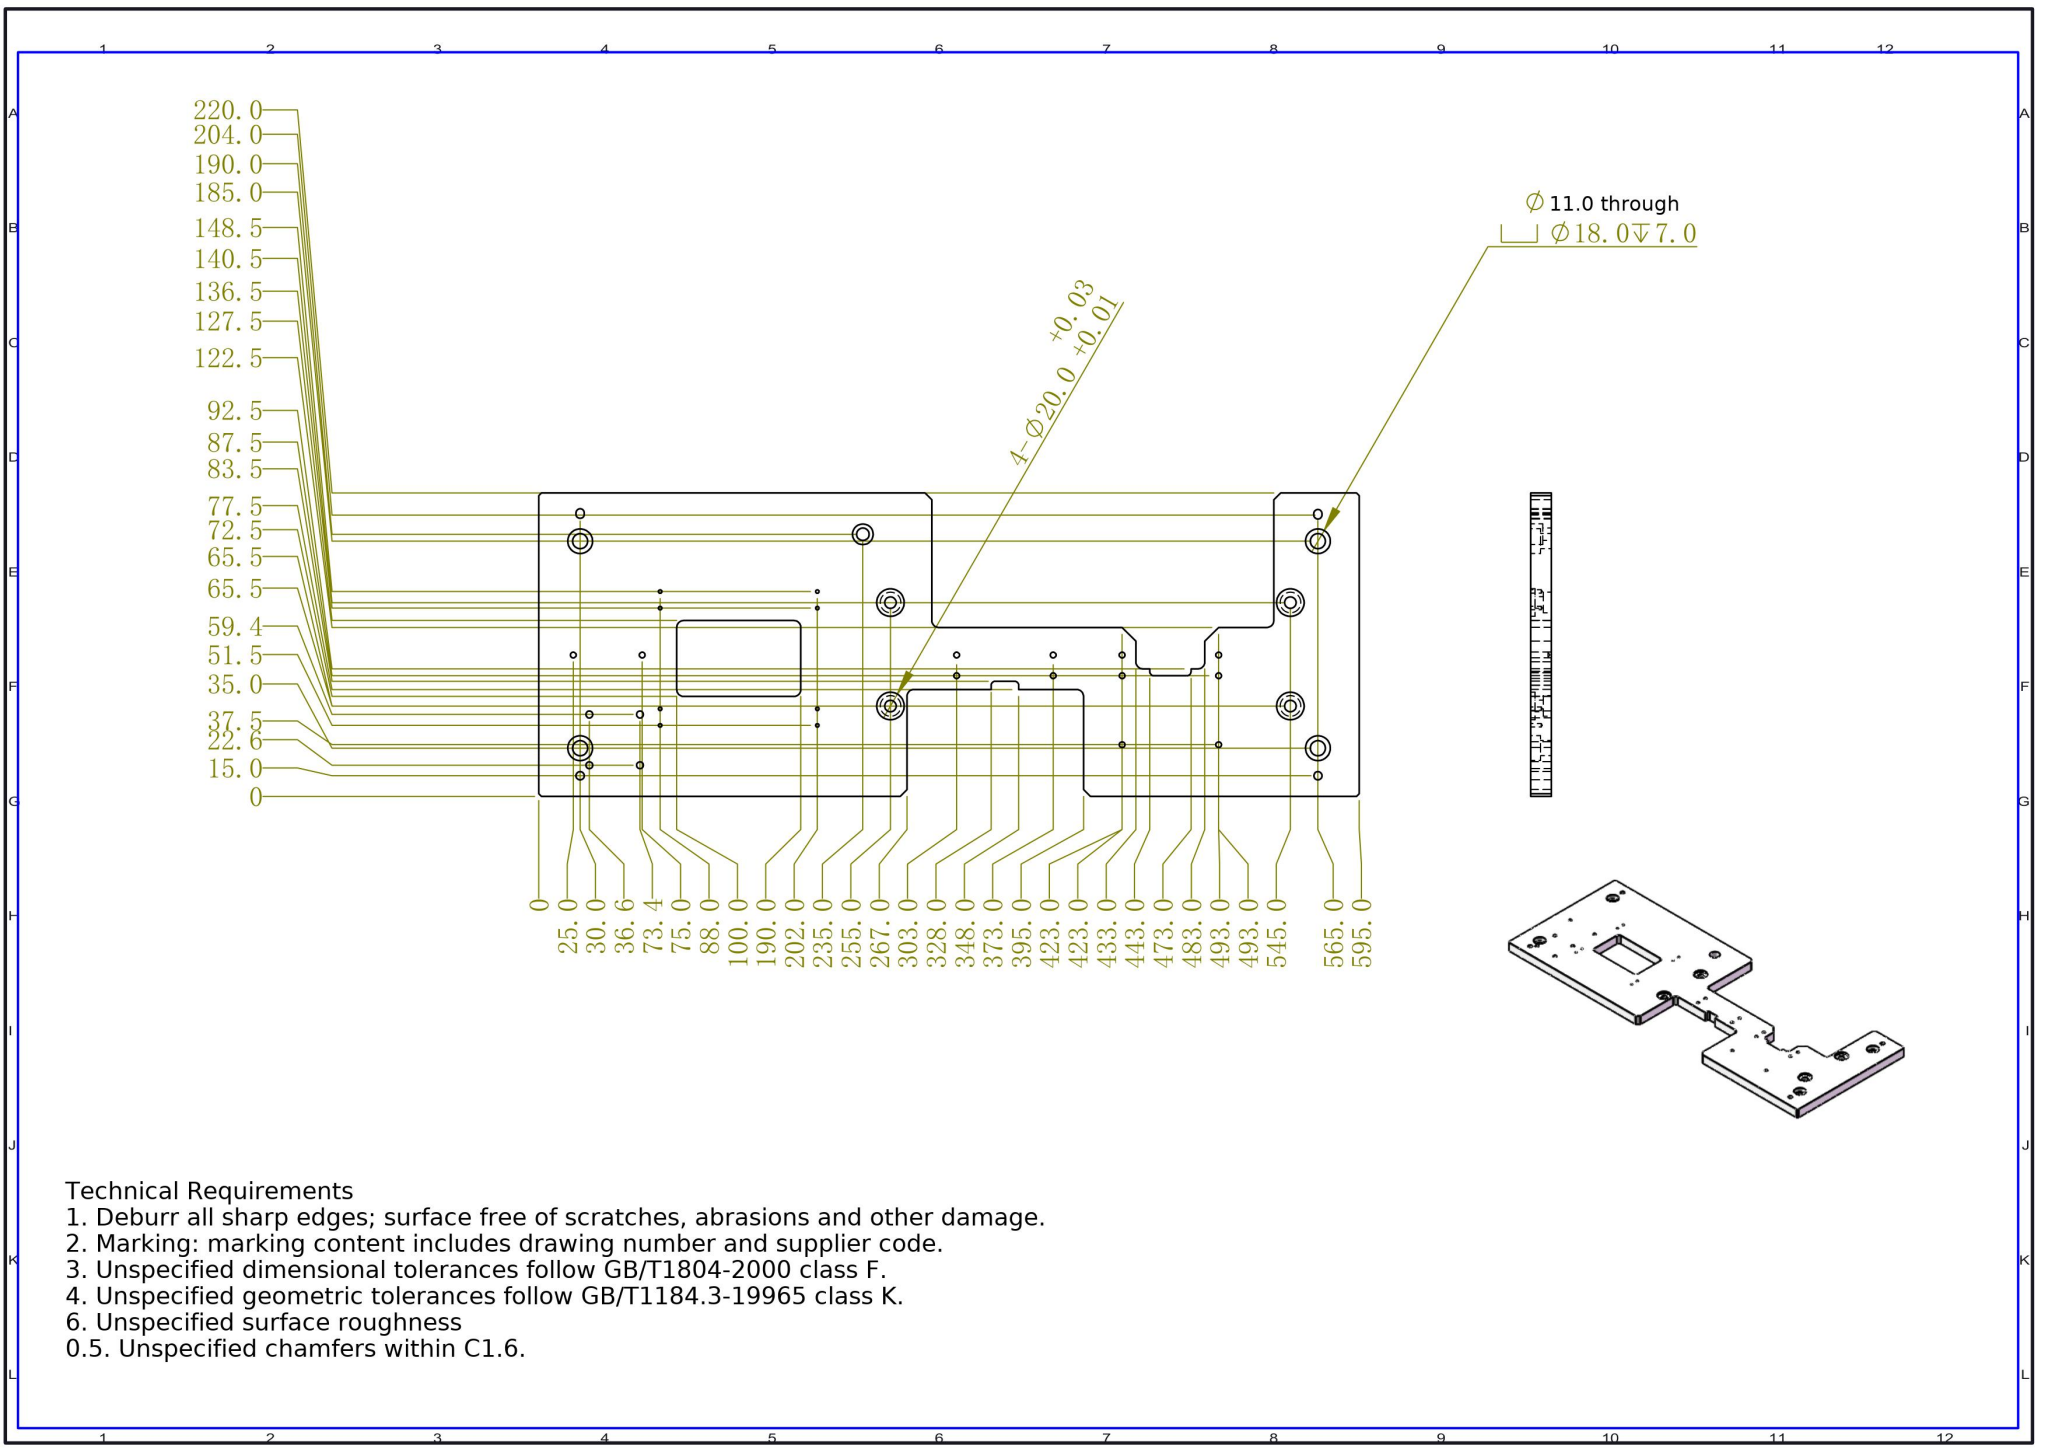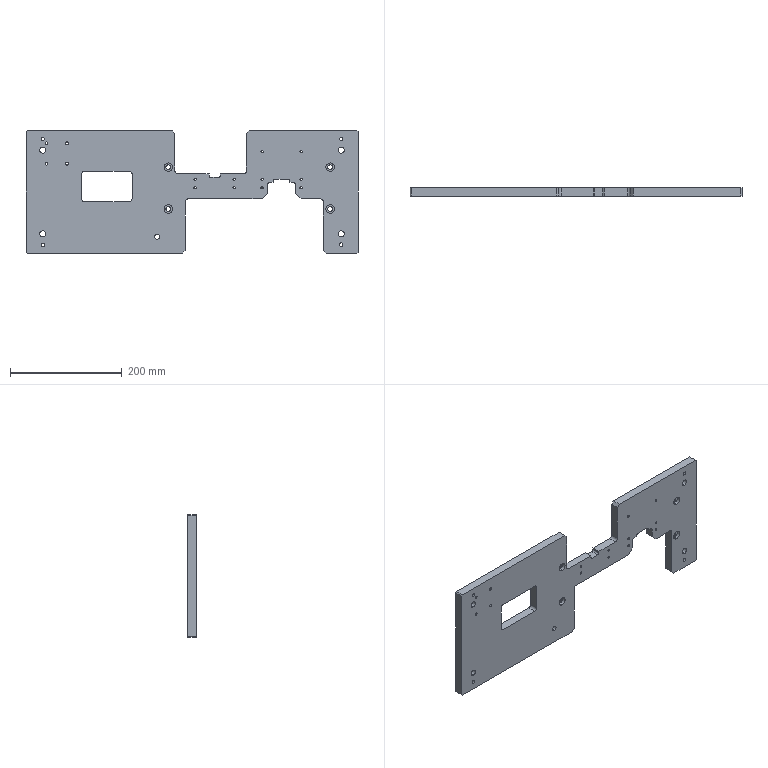Part | SolidWorks | mm | 1 solid | 193 faces | box 595 x 15 x 220 mm | volume 1322563 mm3 | cylinder 116 | plane 57 | cone 20 | commonest cylinder face diameters 2.5 x16 6 x14 4.2 x12 4.134 x12 15 x10 10 x10 5 x8 18 x8